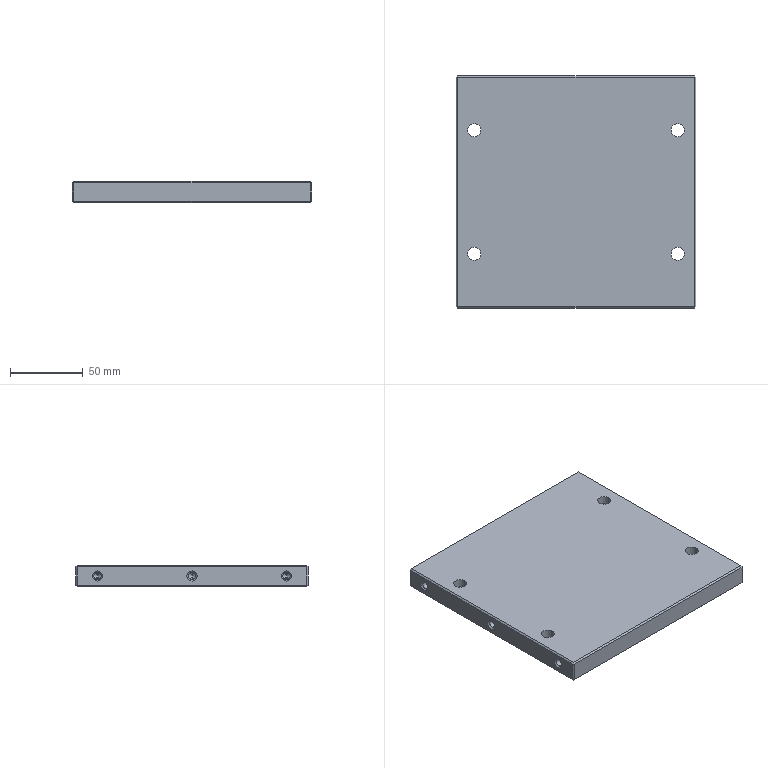Component | SolidWorks | BasePlate2-1 | 1 solid | 82 faces | box 165 x 160 x 15 mm | volume 385557 mm3 | plane 30 | cylinder 28 | cone 24 | commonest cylinder face diameters 5 x12 15 x8 9 x8 | material 1060 Alloy
build123d program:
from build123d import *

# Parameters (mm, degrees)
SKETCH1_W                                          = 165
SKETCH1_H                                          = 160
BOSS_EXTRUDE1_DEPTH                                = 7.5
M6_TAPPED_HOLE1_D                                  = 5
M6_TAPPED_HOLE1_DEPTH                              = 15
M6_TAPPED_HOLE1_TIP                                = 1.502
M6_TAPPED_HOLE2_D                                  = 5
M6_TAPPED_HOLE2_DEPTH                              = 15
M6_TAPPED_HOLE2_TIP                                = 1.502
CHAMFER1_SIZE                                      = 1
HOLE_SIZE_ACCORDING_TO_TYPE_OF_HEXAGON_D           = 9
HOLE_SIZE_ACCORDING_TO_TYPE_OF_HEXAGON_CBORE_D     = 15
HOLE_SIZE_ACCORDING_TO_TYPE_OF_HEXAGON_CBORE_DEPTH = 9


with BuildPart() as part:
    # Sketch1 → Boss-Extrude1 (new, symmetric)
    with BuildSketch(Plane.XY):
        Rectangle(SKETCH1_W, SKETCH1_H)
    extrude(amount=BOSS_EXTRUDE1_DEPTH, both=True)

    # M6 Tapped Hole1
    with Locations(Plane.ZY.offset(82.5)):
        with Locations((0, 0), (0, 65), (0, -65)):
            Hole(M6_TAPPED_HOLE1_D / 2, depth=M6_TAPPED_HOLE1_DEPTH)
            with Locations((0, 0, -(M6_TAPPED_HOLE1_DEPTH + M6_TAPPED_HOLE1_TIP / 2))):  # 118° drill point
                Cone(0, M6_TAPPED_HOLE1_D / 2, M6_TAPPED_HOLE1_TIP, mode=Mode.SUBTRACT)

    # M6 Tapped Hole2
    with Locations(Plane(origin=(82.5, 0, 0), x_dir=(0, 0, -1), z_dir=(1, 0, 0))):
        with Locations((0, 65), (0, 0), (0, -65)):
            Hole(M6_TAPPED_HOLE2_D / 2, depth=M6_TAPPED_HOLE2_DEPTH)
            with Locations((0, 0, -(M6_TAPPED_HOLE2_DEPTH + M6_TAPPED_HOLE2_TIP / 2))):  # 118° drill point
                Cone(0, M6_TAPPED_HOLE2_D / 2, M6_TAPPED_HOLE2_TIP, mode=Mode.SUBTRACT)

    # Chamfer1
    chamfer1_edges = [part.edges().sort_by_distance(p)[0] for p in [
        (82.5, 0, 7.5),
        (0, 80, 7.5),
        (-82.5, -65, 2.5),
        (-82.5, 65, 2.5),
        (-82.5, 0, 2.5),
        (82.5, -65, -2.5),
        (82.5, 0, -2.5),
        (82.5, 65, -2.5),
        (-82.5, 0, 7.5),
        (0, 80, -7.5),
        (82.5, 0, -7.5),
        (0, -80, -7.5),
        (-82.5, 0, -7.5),
        (0, -80, 7.5),
        (-82.5, 80, 0),
        (82.5, 80, 0),
        (82.5, -80, 0),
        (-82.5, -80, 0),
    ]]
    chamfer(chamfer1_edges, length=CHAMFER1_SIZE)

    # Hole Size _according to_ type of Hexagon (through all)
    with Locations(Plane(origin=(0, 0, -7.5), x_dir=(-1, 0, 0), z_dir=(0, 0, -1))):
        with Locations((-70, 42.5), (70, 42.5), (70, -42.5), (-70, -42.5)):
            CounterBoreHole(HOLE_SIZE_ACCORDING_TO_TYPE_OF_HEXAGON_D / 2, HOLE_SIZE_ACCORDING_TO_TYPE_OF_HEXAGON_CBORE_D / 2, HOLE_SIZE_ACCORDING_TO_TYPE_OF_HEXAGON_CBORE_DEPTH)


solid = part.part

# Placed as in the assembly
solid = solid.moved(Location((-47.166, 40.264, 190), (0, 0, 0)))